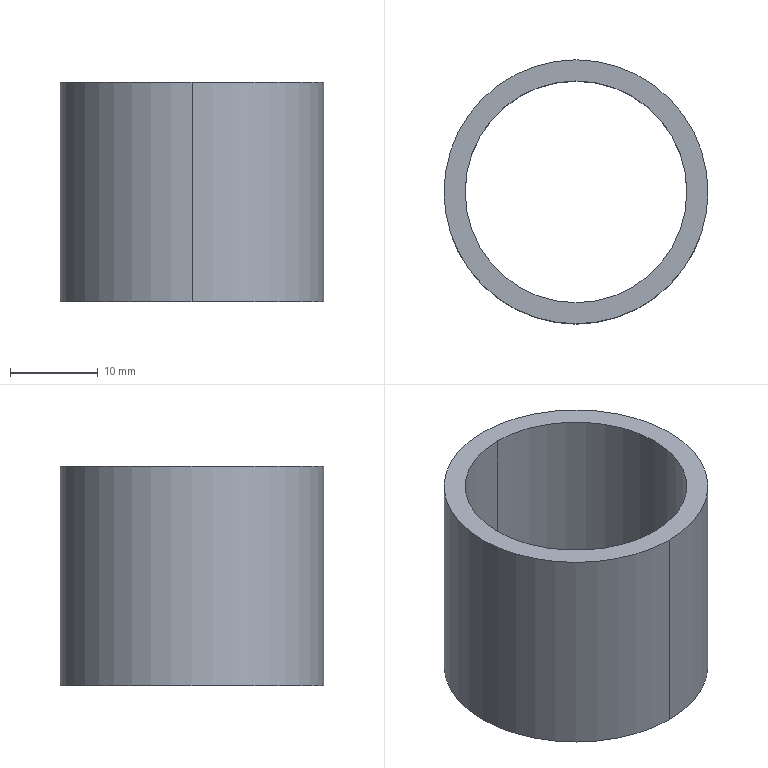Component | SolidWorks | TractionDriveWheelAssembly-1_TractionDriveWheelLimitSleeve-1 | 1 solid | 6 faces | box 30 x 30 x 25 mm | volume 5202 mm3 | cylinder 4 | plane 2 | commonest cylinder face diameters 25.2 x2 30 x2
build123d program:
from build123d import *

# Parameters (mm, degrees)
SKETCH1_R           = 15
SKETCH1_R_2         = 12.6
BOSS_EXTRUDE1_DEPTH = 12.5


with BuildPart() as part:
    # Sketch1 → Boss-Extrude1 (new, symmetric)
    with BuildSketch(Plane.XY):
        Circle(SKETCH1_R)
        Circle(SKETCH1_R_2, mode=Mode.SUBTRACT)
    extrude(amount=BOSS_EXTRUDE1_DEPTH, both=True)


solid = part.part

# Placed as in the assembly
solid = solid.moved(Location((-299.507, -39.911, 507.5), (0, 0, 0)))
STEP:
#1=COLOUR_RGB('',0.7922,0.8196,0.9333);
#2=FILL_AREA_STYLE_COLOUR('',#1);
#3=FILL_AREA_STYLE('',(#2));
#4=SURFACE_STYLE_FILL_AREA(#3);
#5=SURFACE_SIDE_STYLE('',(#4));
#6=SURFACE_STYLE_USAGE(.BOTH.,#5);
#7=PRESENTATION_STYLE_ASSIGNMENT((#6));
#8=CARTESIAN_POINT('',(-11.792,-2.067,20.472));
#9=VERTEX_POINT('',#8);
#10=CARTESIAN_POINT('',(-11.792,-1.075,20.472));
#11=VERTEX_POINT('',#10);
#12=CARTESIAN_POINT('',(-11.792,-1.571,20.472));
#13=DIRECTION('',(-0.,-0.,1.));
#14=DIRECTION('',(-0.,1.,0.));
#15=AXIS2_PLACEMENT_3D('',#12,#13,#14);
#16=CIRCLE('',#15,0.4961);
#17=EDGE_CURVE('',#9,#11,#16,.T.);
#18=ORIENTED_EDGE('',*,*,#17,.T.);
#19=CARTESIAN_POINT('',(-11.792,-1.075,19.488));
#20=VERTEX_POINT('',#19);
#21=CARTESIAN_POINT('',(-11.792,-1.075,20.472));
#22=DIRECTION('',(0.,0.,-1.));
#23=VECTOR('',#22,39.37);
#24=LINE('',#21,#23);
#25=EDGE_CURVE('',#11,#20,#24,.T.);
#26=ORIENTED_EDGE('',*,*,#25,.T.);
#27=CARTESIAN_POINT('',(-11.792,-2.067,19.488));
#28=VERTEX_POINT('',#27);
#29=CARTESIAN_POINT('',(-11.792,-1.571,19.488));
#30=DIRECTION('',(-0.,-0.,1.));
#31=DIRECTION('',(-0.,1.,0.));
#32=AXIS2_PLACEMENT_3D('',#29,#30,#31);
#33=CIRCLE('',#32,0.4961);
#34=EDGE_CURVE('',#28,#20,#33,.T.);
#35=ORIENTED_EDGE('',*,*,#34,.F.);
#36=CARTESIAN_POINT('',(-11.792,-2.067,20.472));
#37=DIRECTION('',(0.,0.,-1.));
#38=VECTOR('',#37,39.37);
#39=LINE('',#36,#38);
#40=EDGE_CURVE('',#9,#28,#39,.T.);
#41=ORIENTED_EDGE('',*,*,#40,.F.);
#42=EDGE_LOOP('',(#18,#26,#35,#41));
#43=FACE_OUTER_BOUND('',#42,.T.);
#44=CARTESIAN_POINT('',(-11.792,-1.571,20.472));
#45=DIRECTION('',(0.,0.,-1.));
#46=DIRECTION('',(0.,-1.,0.));
#47=AXIS2_PLACEMENT_3D('',#44,#45,#46);
#48=CYLINDRICAL_SURFACE('',#47,0.4961);
#49=ADVANCED_FACE('',(#43),#48,.F.);
#50=CARTESIAN_POINT('',(-11.792,-0.9808,20.472));
#51=VERTEX_POINT('',#50);
#52=CARTESIAN_POINT('',(-11.792,-2.162,20.472));
#53=VERTEX_POINT('',#52);
#54=CARTESIAN_POINT('',(-11.792,-1.571,20.472));
#55=DIRECTION('',(-0.,-0.,1.));
#56=DIRECTION('',(-0.,1.,0.));
#57=AXIS2_PLACEMENT_3D('',#54,#55,#56);
#58=CIRCLE('',#57,0.5906);
#59=EDGE_CURVE('',#51,#53,#58,.T.);
#60=ORIENTED_EDGE('',*,*,#59,.F.);
#61=CARTESIAN_POINT('',(-11.792,-0.9808,19.488));
#62=VERTEX_POINT('',#61);
#63=CARTESIAN_POINT('',(-11.792,-0.9808,20.472));
#64=DIRECTION('',(0.,0.,-1.));
#65=VECTOR('',#64,39.37);
#66=LINE('',#63,#65);
#67=EDGE_CURVE('',#51,#62,#66,.T.);
#68=ORIENTED_EDGE('',*,*,#67,.T.);
#69=CARTESIAN_POINT('',(-11.792,-2.162,19.488));
#70=VERTEX_POINT('',#69);
#71=CARTESIAN_POINT('',(-11.792,-1.571,19.488));
#72=DIRECTION('',(-0.,-0.,1.));
#73=DIRECTION('',(-0.,1.,0.));
#74=AXIS2_PLACEMENT_3D('',#71,#72,#73);
#75=CIRCLE('',#74,0.5906);
#76=EDGE_CURVE('',#62,#70,#75,.T.);
#77=ORIENTED_EDGE('',*,*,#76,.T.);
#78=CARTESIAN_POINT('',(-11.792,-2.162,20.472));
#79=DIRECTION('',(0.,0.,-1.));
#80=VECTOR('',#79,39.37);
#81=LINE('',#78,#80);
#82=EDGE_CURVE('',#53,#70,#81,.T.);
#83=ORIENTED_EDGE('',*,*,#82,.F.);
#84=EDGE_LOOP('',(#60,#68,#77,#83));
#85=FACE_OUTER_BOUND('',#84,.T.);
#86=CARTESIAN_POINT('',(-11.792,-1.571,20.472));
#87=DIRECTION('',(0.,0.,-1.));
#88=DIRECTION('',(0.,-1.,0.));
#89=AXIS2_PLACEMENT_3D('',#86,#87,#88);
#90=CYLINDRICAL_SURFACE('',#89,0.5906);
#91=ADVANCED_FACE('',(#85),#90,.T.);
#92=CARTESIAN_POINT('',(-11.792,-1.571,20.472));
#93=DIRECTION('',(-0.,-0.,1.));
#94=DIRECTION('',(-0.,1.,0.));
#95=AXIS2_PLACEMENT_3D('',#92,#93,#94);
#96=CIRCLE('',#95,0.5906);
#97=EDGE_CURVE('',#53,#51,#96,.T.);
#98=ORIENTED_EDGE('',*,*,#97,.T.);
#99=ORIENTED_EDGE('',*,*,#59,.T.);
#100=EDGE_LOOP('',(#98,#99));
#101=FACE_OUTER_BOUND('',#100,.T.);
#102=ORIENTED_EDGE('',*,*,#17,.F.);
#103=CARTESIAN_POINT('',(-11.792,-1.571,20.472));
#104=DIRECTION('',(-0.,-0.,1.));
#105=DIRECTION('',(-0.,1.,0.));
#106=AXIS2_PLACEMENT_3D('',#103,#104,#105);
#107=CIRCLE('',#106,0.4961);
#108=EDGE_CURVE('',#11,#9,#107,.T.);
#109=ORIENTED_EDGE('',*,*,#108,.F.);
#110=EDGE_LOOP('',(#102,#109));
#111=FACE_BOUND('',#110,.T.);
#112=CARTESIAN_POINT('',(-11.792,-1.571,20.472));
#113=DIRECTION('',(-0.,-0.,1.));
#114=DIRECTION('',(-0.,1.,0.));
#115=AXIS2_PLACEMENT_3D('',#112,#113,#114);
#116=PLANE('',#115);
#117=ADVANCED_FACE('',(#101,#111),#116,.T.);
#118=CARTESIAN_POINT('',(-11.792,-1.571,19.488));
#119=DIRECTION('',(-0.,-0.,1.));
#120=DIRECTION('',(-0.,1.,0.));
#121=AXIS2_PLACEMENT_3D('',#118,#119,#120);
#122=CIRCLE('',#121,0.5906);
#123=EDGE_CURVE('',#70,#62,#122,.T.);
#124=ORIENTED_EDGE('',*,*,#123,.F.);
#125=ORIENTED_EDGE('',*,*,#76,.F.);
#126=EDGE_LOOP('',(#124,#125));
#127=FACE_OUTER_BOUND('',#126,.T.);
#128=ORIENTED_EDGE('',*,*,#34,.T.);
#129=CARTESIAN_POINT('',(-11.792,-1.571,19.488));
#130=DIRECTION('',(-0.,-0.,1.));
#131=DIRECTION('',(-0.,1.,0.));
#132=AXIS2_PLACEMENT_3D('',#129,#130,#131);
#133=CIRCLE('',#132,0.4961);
#134=EDGE_CURVE('',#20,#28,#133,.T.);
#135=ORIENTED_EDGE('',*,*,#134,.T.);
#136=EDGE_LOOP('',(#128,#135));
#137=FACE_BOUND('',#136,.T.);
#138=CARTESIAN_POINT('',(-11.792,-1.571,19.488));
#139=DIRECTION('',(-0.,-0.,1.));
#140=DIRECTION('',(-0.,1.,0.));
#141=AXIS2_PLACEMENT_3D('',#138,#139,#140);
#142=PLANE('',#141);
#143=ADVANCED_FACE('',(#127,#137),#142,.F.);
#144=ORIENTED_EDGE('',*,*,#67,.F.);
#145=ORIENTED_EDGE('',*,*,#97,.F.);
#146=ORIENTED_EDGE('',*,*,#82,.T.);
#147=ORIENTED_EDGE('',*,*,#123,.T.);
#148=EDGE_LOOP('',(#144,#145,#146,#147));
#149=FACE_OUTER_BOUND('',#148,.T.);
#150=CARTESIAN_POINT('',(-11.792,-1.571,20.472));
#151=DIRECTION('',(0.,0.,-1.));
#152=DIRECTION('',(0.,-1.,0.));
#153=AXIS2_PLACEMENT_3D('',#150,#151,#152);
#154=CYLINDRICAL_SURFACE('',#153,0.5906);
#155=ADVANCED_FACE('',(#149),#154,.T.);
#156=ORIENTED_EDGE('',*,*,#25,.F.);
#157=ORIENTED_EDGE('',*,*,#108,.T.);
#158=ORIENTED_EDGE('',*,*,#40,.T.);
#159=ORIENTED_EDGE('',*,*,#134,.F.);
#160=EDGE_LOOP('',(#156,#157,#158,#159));
#161=FACE_OUTER_BOUND('',#160,.T.);
#162=CARTESIAN_POINT('',(-11.792,-1.571,20.472));
#163=DIRECTION('',(0.,0.,-1.));
#164=DIRECTION('',(0.,-1.,0.));
#165=AXIS2_PLACEMENT_3D('',#162,#163,#164);
#166=CYLINDRICAL_SURFACE('',#165,0.4961);
#167=ADVANCED_FACE('',(#161),#166,.F.);
#168=CLOSED_SHELL('',(#49,#91,#117,#143,#155,#167));
#169=MANIFOLD_SOLID_BREP('',#168);
#170=STYLED_ITEM('',(#7),#169);
#171=(LENGTH_UNIT()NAMED_UNIT(*)SI_UNIT($,.METRE.));
#172=LENGTH_MEASURE_WITH_UNIT(LENGTH_MEASURE(0.0254),#171);
#173=DIMENSIONAL_EXPONENTS(1.,0.,0.,0.,0.,0.,0.);
#174=(CONVERSION_BASED_UNIT('',#172)LENGTH_UNIT()NAMED_UNIT(#173));
#175=UNCERTAINTY_MEASURE_WITH_UNIT(LENGTH_MEASURE(0.00001),#174,'','');
#176=(NAMED_UNIT(*)PLANE_ANGLE_UNIT()SI_UNIT($,.RADIAN.));
#177=(NAMED_UNIT(*)SI_UNIT($,.STERADIAN.)SOLID_ANGLE_UNIT());
#178=(GEOMETRIC_REPRESENTATION_CONTEXT(3)GLOBAL_UNCERTAINTY_ASSIGNED_CONTEXT((#175))GLOBAL_UNIT_ASSIGNED_CONTEXT((#174,#176,#177))REPRESENTATION_CONTEXT('',''));
#179=MECHANICAL_DESIGN_GEOMETRIC_PRESENTATION_REPRESENTATION('',(#170),#178);
#180=PRESENTATION_LAYER_ASSIGNMENT('','',(#170));
#181=CARTESIAN_POINT('',(0.,0.,0.));
#182=DIRECTION('',(0.,0.,1.));
#183=DIRECTION('',(1.,0.,0.));
#184=AXIS2_PLACEMENT_3D('',#181,#182,#183);
#185=(LENGTH_UNIT()NAMED_UNIT(*)SI_UNIT($,.METRE.));
#186=LENGTH_MEASURE_WITH_UNIT(LENGTH_MEASURE(0.0254),#185);
#187=DIMENSIONAL_EXPONENTS(1.,0.,0.,0.,0.,0.,0.);
#188=(CONVERSION_BASED_UNIT('',#186)LENGTH_UNIT()NAMED_UNIT(#187));
#189=UNCERTAINTY_MEASURE_WITH_UNIT(LENGTH_MEASURE(0.00001),#188,'','');
#190=(NAMED_UNIT(*)PLANE_ANGLE_UNIT()SI_UNIT($,.RADIAN.));
#191=(NAMED_UNIT(*)SI_UNIT($,.STERADIAN.)SOLID_ANGLE_UNIT());
#192=(GEOMETRIC_REPRESENTATION_CONTEXT(3)GLOBAL_UNCERTAINTY_ASSIGNED_CONTEXT((#189))GLOBAL_UNIT_ASSIGNED_CONTEXT((#188,#190,#191))REPRESENTATION_CONTEXT('',''));
#193=ADVANCED_BREP_SHAPE_REPRESENTATION('',(#169,#184),#192);